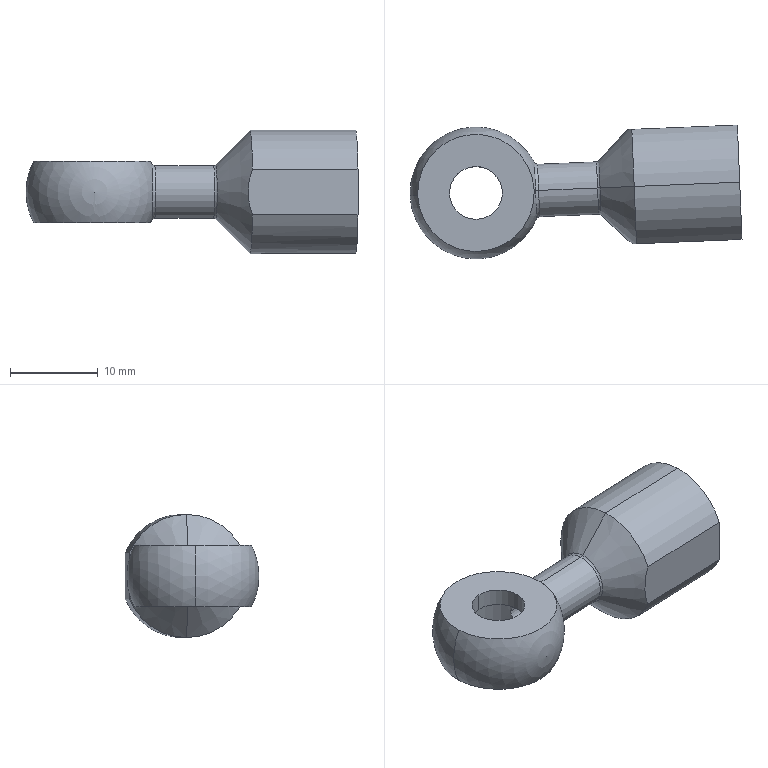Component | SolidWorks | 6.11-1937032106-0-2 | 1 solid | 33 faces | box 37.74 x 15.21 x 14 mm | volume 2451 mm3 | cylinder 16 | plane 7 | torus 4 | cone 4 | sphere 2 | commonest cylinder face diameters 6 x6 8 x3 14 x3 8.8 x2 3 x2 | material 40Cr
STEP:
#1=COLOUR_RGB('',0.7922,0.8196,0.9333);
#2=FILL_AREA_STYLE_COLOUR('',#1);
#3=FILL_AREA_STYLE('',(#2));
#4=SURFACE_STYLE_FILL_AREA(#3);
#5=SURFACE_SIDE_STYLE('',(#4));
#6=SURFACE_STYLE_USAGE(.BOTH.,#5);
#7=PRESENTATION_STYLE_ASSIGNMENT((#6));
#8=CARTESIAN_POINT('',(0.2663,-1.761,-2.076));
#9=VERTEX_POINT('',#8);
#10=CARTESIAN_POINT('',(0.2663,-1.761,-1.822));
#11=VERTEX_POINT('',#10);
#12=CARTESIAN_POINT('',(0.2663,-1.761,-1.949));
#13=DIRECTION('',(-0.9992,-0.0406,0.));
#14=DIRECTION('',(0.,0.,1.));
#15=AXIS2_PLACEMENT_3D('',#12,#13,#14);
#16=CIRCLE('',#15,0.1271);
#17=EDGE_CURVE('',#9,#11,#16,.T.);
#18=ORIENTED_EDGE('',*,*,#17,.F.);
#19=CARTESIAN_POINT('',(0.2805,-1.76,-2.067));
#20=VERTEX_POINT('',#19);
#21=CARTESIAN_POINT('',(0.2805,-1.76,-2.083));
#22=DIRECTION('',(-0.0406,0.9992,0.));
#23=DIRECTION('',(-0.9992,-0.0406,0.));
#24=AXIS2_PLACEMENT_3D('',#21,#22,#23);
#25=CIRCLE('',#24,0.01575);
#26=EDGE_CURVE('',#9,#20,#25,.T.);
#27=ORIENTED_EDGE('',*,*,#26,.T.);
#28=CARTESIAN_POINT('',(0.2805,-1.76,-1.831));
#29=VERTEX_POINT('',#28);
#30=CARTESIAN_POINT('',(0.2805,-1.76,-1.949));
#31=DIRECTION('',(0.9992,0.0406,-0.));
#32=DIRECTION('',(0.,0.,1.));
#33=AXIS2_PLACEMENT_3D('',#30,#31,#32);
#34=CIRCLE('',#33,0.1181);
#35=EDGE_CURVE('',#29,#20,#34,.T.);
#36=ORIENTED_EDGE('',*,*,#35,.F.);
#37=CARTESIAN_POINT('',(0.2805,-1.76,-1.815));
#38=DIRECTION('',(0.0406,-0.9992,0.));
#39=DIRECTION('',(0.9992,0.0406,0.));
#40=AXIS2_PLACEMENT_3D('',#37,#38,#39);
#41=CIRCLE('',#40,0.01575);
#42=EDGE_CURVE('',#11,#29,#41,.T.);
#43=ORIENTED_EDGE('',*,*,#42,.F.);
#44=EDGE_LOOP('',(#18,#27,#36,#43));
#45=FACE_OUTER_BOUND('',#44,.T.);
#46=CARTESIAN_POINT('',(0.2805,-1.76,-1.949));
#47=DIRECTION('',(-0.9992,-0.0406,0.));
#48=DIRECTION('',(0.,-0.,1.));
#49=AXIS2_PLACEMENT_3D('',#46,#47,#48);
#50=TOROIDAL_SURFACE('',#49,0.1339,0.01575);
#51=ADVANCED_FACE('',(#45),#50,.F.);
#52=CARTESIAN_POINT('',(0.5442,-1.75,-2.067));
#53=VERTEX_POINT('',#52);
#54=CARTESIAN_POINT('',(0.5442,-1.75,-1.831));
#55=VERTEX_POINT('',#54);
#56=CARTESIAN_POINT('',(0.5442,-1.75,-1.949));
#57=DIRECTION('',(-0.9992,-0.0406,0.));
#58=DIRECTION('',(0.,0.,1.));
#59=AXIS2_PLACEMENT_3D('',#56,#57,#58);
#60=CIRCLE('',#59,0.1181);
#61=EDGE_CURVE('',#53,#55,#60,.T.);
#62=ORIENTED_EDGE('',*,*,#61,.F.);
#63=CARTESIAN_POINT('',(0.5553,-1.749,-2.072));
#64=VERTEX_POINT('',#63);
#65=CARTESIAN_POINT('',(0.5442,-1.75,-2.083));
#66=DIRECTION('',(-0.0406,0.9992,0.));
#67=DIRECTION('',(-0.9992,-0.0406,0.));
#68=AXIS2_PLACEMENT_3D('',#65,#66,#67);
#69=CIRCLE('',#68,0.01575);
#70=EDGE_CURVE('',#53,#64,#69,.T.);
#71=ORIENTED_EDGE('',*,*,#70,.T.);
#72=CARTESIAN_POINT('',(0.5553,-1.749,-1.826));
#73=VERTEX_POINT('',#72);
#74=CARTESIAN_POINT('',(0.5553,-1.749,-1.949));
#75=DIRECTION('',(0.9992,0.0406,-0.));
#76=DIRECTION('',(0.,0.,-1.));
#77=AXIS2_PLACEMENT_3D('',#74,#75,#76);
#78=CIRCLE('',#77,0.1227);
#79=EDGE_CURVE('',#73,#64,#78,.T.);
#80=ORIENTED_EDGE('',*,*,#79,.F.);
#81=CARTESIAN_POINT('',(0.5442,-1.75,-1.815));
#82=DIRECTION('',(0.0406,-0.9992,0.));
#83=DIRECTION('',(0.9992,0.0406,0.));
#84=AXIS2_PLACEMENT_3D('',#81,#82,#83);
#85=CIRCLE('',#84,0.01575);
#86=EDGE_CURVE('',#55,#73,#85,.T.);
#87=ORIENTED_EDGE('',*,*,#86,.F.);
#88=EDGE_LOOP('',(#62,#71,#80,#87));
#89=FACE_OUTER_BOUND('',#88,.T.);
#90=CARTESIAN_POINT('',(0.5442,-1.75,-1.949));
#91=DIRECTION('',(-0.9992,-0.0406,0.));
#92=DIRECTION('',(0.,0.,1.));
#93=AXIS2_PLACEMENT_3D('',#90,#91,#92);
#94=TOROIDAL_SURFACE('',#93,0.1339,0.01575);
#95=ADVANCED_FACE('',(#89),#94,.F.);
#96=CARTESIAN_POINT('',(0.006394,-1.929,-1.89));
#97=VERTEX_POINT('',#96);
#98=CARTESIAN_POINT('',(-0.006394,-1.614,-1.89));
#99=VERTEX_POINT('',#98);
#100=CARTESIAN_POINT('',(0.,-1.772,-1.89));
#101=DIRECTION('',(0.,0.,-1.));
#102=DIRECTION('',(-0.0406,0.9992,0.));
#103=AXIS2_PLACEMENT_3D('',#100,#101,#102);
#104=CIRCLE('',#103,0.1575);
#105=EDGE_CURVE('',#97,#99,#104,.T.);
#106=ORIENTED_EDGE('',*,*,#105,.F.);
#107=CARTESIAN_POINT('',(0.006394,-1.929,-2.008));
#108=VERTEX_POINT('',#107);
#109=CARTESIAN_POINT('',(0.006394,-1.929,-1.89));
#110=DIRECTION('',(0.,0.,-1.));
#111=VECTOR('',#110,39.37);
#112=LINE('',#109,#111);
#113=EDGE_CURVE('',#97,#108,#112,.T.);
#114=ORIENTED_EDGE('',*,*,#113,.T.);
#115=CARTESIAN_POINT('',(-0.006394,-1.614,-2.008));
#116=VERTEX_POINT('',#115);
#117=CARTESIAN_POINT('',(0.,-1.772,-2.008));
#118=DIRECTION('',(0.,0.,-1.));
#119=DIRECTION('',(-0.0406,0.9992,0.));
#120=AXIS2_PLACEMENT_3D('',#117,#118,#119);
#121=CIRCLE('',#120,0.1575);
#122=EDGE_CURVE('',#108,#116,#121,.T.);
#123=ORIENTED_EDGE('',*,*,#122,.T.);
#124=CARTESIAN_POINT('',(-0.006394,-1.614,-1.89));
#125=DIRECTION('',(0.,0.,-1.));
#126=VECTOR('',#125,39.37);
#127=LINE('',#124,#126);
#128=EDGE_CURVE('',#99,#116,#127,.T.);
#129=ORIENTED_EDGE('',*,*,#128,.F.);
#130=EDGE_LOOP('',(#106,#114,#123,#129));
#131=FACE_OUTER_BOUND('',#130,.T.);
#132=CARTESIAN_POINT('',(0.,-1.772,-1.89));
#133=DIRECTION('',(0.,0.,-1.));
#134=DIRECTION('',(-0.0406,0.9992,0.));
#135=AXIS2_PLACEMENT_3D('',#132,#133,#134);
#136=CYLINDRICAL_SURFACE('',#135,0.1575);
#137=ADVANCED_FACE('',(#131),#136,.F.);
#138=CARTESIAN_POINT('',(0.1574,-1.765,-1.89));
#139=VERTEX_POINT('',#138);
#140=CARTESIAN_POINT('',(0.,-1.772,-1.89));
#141=DIRECTION('',(0.,0.,-1.));
#142=DIRECTION('',(-0.0406,0.9992,0.));
#143=AXIS2_PLACEMENT_3D('',#140,#141,#142);
#144=CIRCLE('',#143,0.1575);
#145=EDGE_CURVE('',#99,#139,#144,.T.);
#146=ORIENTED_EDGE('',*,*,#145,.F.);
#147=ORIENTED_EDGE('',*,*,#128,.T.);
#148=CARTESIAN_POINT('',(0.1574,-1.765,-2.008));
#149=VERTEX_POINT('',#148);
#150=CARTESIAN_POINT('',(0.,-1.772,-2.008));
#151=DIRECTION('',(0.,0.,-1.));
#152=DIRECTION('',(-0.0406,0.9992,0.));
#153=AXIS2_PLACEMENT_3D('',#150,#151,#152);
#154=CIRCLE('',#153,0.1575);
#155=EDGE_CURVE('',#116,#149,#154,.T.);
#156=ORIENTED_EDGE('',*,*,#155,.T.);
#157=CARTESIAN_POINT('',(0.1435,-1.707,-1.949));
#158=VERTEX_POINT('',#157);
#159=CARTESIAN_POINT('',(0.1435,-1.707,-1.949));
#160=CARTESIAN_POINT('',(0.1435,-1.707,-1.957));
#161=CARTESIAN_POINT('',(0.1442,-1.708,-1.964));
#162=CARTESIAN_POINT('',(0.146,-1.713,-1.975));
#163=CARTESIAN_POINT('',(0.1467,-1.714,-1.979));
#164=CARTESIAN_POINT('',(0.1483,-1.719,-1.985));
#165=CARTESIAN_POINT('',(0.1492,-1.721,-1.988));
#166=CARTESIAN_POINT('',(0.1517,-1.729,-1.996));
#167=CARTESIAN_POINT('',(0.1535,-1.736,-2.));
#168=CARTESIAN_POINT('',(0.1554,-1.746,-2.005));
#169=CARTESIAN_POINT('',(0.156,-1.75,-2.006));
#170=CARTESIAN_POINT('',(0.1569,-1.757,-2.007));
#171=CARTESIAN_POINT('',(0.1572,-1.761,-2.008));
#172=CARTESIAN_POINT('',(0.1574,-1.765,-2.008));
#173=B_SPLINE_CURVE_WITH_KNOTS('',3,(#159,#160,#161,#162,#163,#164,#165,#166,#167,#168,#169,#170,#171,#172),.UNSPECIFIED.,.F.,.F.,(4,2,2,2,2,2,4),(0.004733,0.005325,0.00562,0.005916,0.006507,0.006803,0.007099),.UNSPECIFIED.);
#174=EDGE_CURVE('',#158,#149,#173,.T.);
#175=ORIENTED_EDGE('',*,*,#174,.F.);
#176=CARTESIAN_POINT('',(0.1574,-1.765,-1.89));
#177=CARTESIAN_POINT('',(0.1572,-1.761,-1.89));
#178=CARTESIAN_POINT('',(0.1569,-1.757,-1.89));
#179=CARTESIAN_POINT('',(0.156,-1.75,-1.892));
#180=CARTESIAN_POINT('',(0.1554,-1.746,-1.893));
#181=CARTESIAN_POINT('',(0.1541,-1.739,-1.896));
#182=CARTESIAN_POINT('',(0.1533,-1.736,-1.898));
#183=CARTESIAN_POINT('',(0.1517,-1.729,-1.902));
#184=CARTESIAN_POINT('',(0.1509,-1.726,-1.904));
#185=CARTESIAN_POINT('',(0.1492,-1.721,-1.91));
#186=CARTESIAN_POINT('',(0.1483,-1.719,-1.913));
#187=CARTESIAN_POINT('',(0.1467,-1.714,-1.919));
#188=CARTESIAN_POINT('',(0.146,-1.713,-1.923));
#189=CARTESIAN_POINT('',(0.1442,-1.708,-1.933));
#190=CARTESIAN_POINT('',(0.1435,-1.707,-1.941));
#191=CARTESIAN_POINT('',(0.1435,-1.707,-1.949));
#192=B_SPLINE_CURVE_WITH_KNOTS('',3,(#176,#177,#178,#179,#180,#181,#182,#183,#184,#185,#186,#187,#188,#189,#190,#191),.UNSPECIFIED.,.F.,.F.,(4,2,2,2,2,2,2,4),(0.002367,0.002663,0.002959,0.003255,0.00355,0.003846,0.004142,0.004733),.UNSPECIFIED.);
#193=EDGE_CURVE('',#139,#158,#192,.T.);
#194=ORIENTED_EDGE('',*,*,#193,.F.);
#195=EDGE_LOOP('',(#146,#147,#156,#175,#194));
#196=FACE_OUTER_BOUND('',#195,.T.);
#197=CARTESIAN_POINT('',(0.,-1.772,-1.89));
#198=DIRECTION('',(0.,0.,-1.));
#199=DIRECTION('',(-0.0406,0.9992,0.));
#200=AXIS2_PLACEMENT_3D('',#197,#198,#199);
#201=CYLINDRICAL_SURFACE('',#200,0.1575);
#202=ADVANCED_FACE('',(#196),#201,.F.);
#203=CARTESIAN_POINT('',(0.7797,-1.567,-1.949));
#204=VERTEX_POINT('',#203);
#205=CARTESIAN_POINT('',(0.7938,-1.913,-1.949));
#206=VERTEX_POINT('',#205);
#207=CARTESIAN_POINT('',(0.7868,-1.74,-1.949));
#208=DIRECTION('',(0.9992,0.0406,0.));
#209=DIRECTION('',(0.0406,-0.9992,0.));
#210=AXIS2_PLACEMENT_3D('',#207,#208,#209);
#211=CIRCLE('',#210,0.1732);
#212=EDGE_CURVE('',#204,#206,#211,.T.);
#213=ORIENTED_EDGE('',*,*,#212,.F.);
#214=CARTESIAN_POINT('',(1.173,-1.551,-1.949));
#215=VERTEX_POINT('',#214);
#216=CARTESIAN_POINT('',(1.173,-1.551,-1.949));
#217=DIRECTION('',(0.9992,0.0406,0.));
#218=VECTOR('',#217,39.37);
#219=LINE('',#216,#218);
#220=EDGE_CURVE('',#204,#215,#219,.T.);
#221=ORIENTED_EDGE('',*,*,#220,.T.);
#222=CARTESIAN_POINT('',(1.187,-1.897,-1.949));
#223=VERTEX_POINT('',#222);
#224=CARTESIAN_POINT('',(1.18,-1.724,-1.949));
#225=DIRECTION('',(0.9992,0.0406,0.));
#226=DIRECTION('',(0.0406,-0.9992,0.));
#227=AXIS2_PLACEMENT_3D('',#224,#225,#226);
#228=CIRCLE('',#227,0.1732);
#229=EDGE_CURVE('',#215,#223,#228,.T.);
#230=ORIENTED_EDGE('',*,*,#229,.T.);
#231=CARTESIAN_POINT('',(1.187,-1.897,-1.949));
#232=DIRECTION('',(0.9992,0.0406,0.));
#233=VECTOR('',#232,39.37);
#234=LINE('',#231,#233);
#235=EDGE_CURVE('',#206,#223,#234,.T.);
#236=ORIENTED_EDGE('',*,*,#235,.F.);
#237=EDGE_LOOP('',(#213,#221,#230,#236));
#238=FACE_OUTER_BOUND('',#237,.T.);
#239=CARTESIAN_POINT('',(1.18,-1.724,-1.949));
#240=DIRECTION('',(0.9992,0.0406,0.));
#241=DIRECTION('',(0.0406,-0.9992,0.));
#242=AXIS2_PLACEMENT_3D('',#239,#240,#241);
#243=CYLINDRICAL_SURFACE('',#242,0.1732);
#244=ADVANCED_FACE('',(#238),#243,.F.);
#245=CARTESIAN_POINT('',(0.7158,-1.683,-1.949));
#246=VERTEX_POINT('',#245);
#247=CARTESIAN_POINT('',(0.7206,-1.801,-1.949));
#248=VERTEX_POINT('',#247);
#249=CARTESIAN_POINT('',(0.7182,-1.742,-1.949));
#250=DIRECTION('',(0.9992,0.0406,0.));
#251=DIRECTION('',(0.0406,-0.9992,0.));
#252=AXIS2_PLACEMENT_3D('',#249,#250,#251);
#253=CIRCLE('',#252,0.05906);
#254=EDGE_CURVE('',#246,#248,#253,.T.);
#255=ORIENTED_EDGE('',*,*,#254,.F.);
#256=CARTESIAN_POINT('',(0.7797,-1.567,-1.949));
#257=DIRECTION('',(0.4798,0.8774,-0.));
#258=VECTOR('',#257,39.37);
#259=LINE('',#256,#258);
#260=EDGE_CURVE('',#246,#204,#259,.T.);
#261=ORIENTED_EDGE('',*,*,#260,.T.);
#262=ORIENTED_EDGE('',*,*,#212,.T.);
#263=CARTESIAN_POINT('',(0.7938,-1.913,-1.949));
#264=DIRECTION('',(0.5494,-0.8355,0.));
#265=VECTOR('',#264,39.37);
#266=LINE('',#263,#265);
#267=EDGE_CURVE('',#248,#206,#266,.T.);
#268=ORIENTED_EDGE('',*,*,#267,.F.);
#269=EDGE_LOOP('',(#255,#261,#262,#268));
#270=FACE_OUTER_BOUND('',#269,.T.);
#271=CARTESIAN_POINT('',(0.7868,-1.74,-1.949));
#272=DIRECTION('',(0.9992,0.0406,0.));
#273=DIRECTION('',(0.0406,-0.9992,0.));
#274=AXIS2_PLACEMENT_3D('',#271,#272,#273);
#275=CONICAL_SURFACE('',#274,0.1732,1.03);
#276=ADVANCED_FACE('',(#270),#275,.F.);
#277=ORIENTED_EDGE('',*,*,#193,.T.);
#278=CARTESIAN_POINT('',(1.178,-1.665,-1.949));
#279=DIRECTION('',(0.9992,0.0406,0.));
#280=VECTOR('',#279,39.37);
#281=LINE('',#278,#280);
#282=EDGE_CURVE('',#158,#246,#281,.T.);
#283=ORIENTED_EDGE('',*,*,#282,.T.);
#284=ORIENTED_EDGE('',*,*,#254,.T.);
#285=CARTESIAN_POINT('',(0.1483,-1.825,-1.949));
#286=VERTEX_POINT('',#285);
#287=CARTESIAN_POINT('',(1.183,-1.783,-1.949));
#288=DIRECTION('',(0.9992,0.0406,0.));
#289=VECTOR('',#288,39.37);
#290=LINE('',#287,#289);
#291=EDGE_CURVE('',#286,#248,#290,.T.);
#292=ORIENTED_EDGE('',*,*,#291,.F.);
#293=CARTESIAN_POINT('',(0.1483,-1.825,-1.949));
#294=CARTESIAN_POINT('',(0.1483,-1.825,-1.945));
#295=CARTESIAN_POINT('',(0.1484,-1.824,-1.941));
#296=CARTESIAN_POINT('',(0.1489,-1.823,-1.933));
#297=CARTESIAN_POINT('',(0.1494,-1.822,-1.93));
#298=CARTESIAN_POINT('',(0.1508,-1.817,-1.919));
#299=CARTESIAN_POINT('',(0.1522,-1.813,-1.912));
#300=CARTESIAN_POINT('',(0.1547,-1.802,-1.902));
#301=CARTESIAN_POINT('',(0.1559,-1.795,-1.897));
#302=CARTESIAN_POINT('',(0.157,-1.784,-1.893));
#303=CARTESIAN_POINT('',(0.1573,-1.781,-1.892));
#304=CARTESIAN_POINT('',(0.1575,-1.773,-1.89));
#305=CARTESIAN_POINT('',(0.1575,-1.769,-1.89));
#306=CARTESIAN_POINT('',(0.1574,-1.765,-1.89));
#307=B_SPLINE_CURVE_WITH_KNOTS('',3,(#293,#294,#295,#296,#297,#298,#299,#300,#301,#302,#303,#304,#305,#306),.UNSPECIFIED.,.F.,.F.,(4,2,2,2,2,2,4),(0.,0.0002959,0.0005918,0.001184,0.001775,0.002071,0.002367),.UNSPECIFIED.);
#308=EDGE_CURVE('',#286,#139,#307,.T.);
#309=ORIENTED_EDGE('',*,*,#308,.T.);
#310=EDGE_LOOP('',(#277,#283,#284,#292,#309));
#311=FACE_OUTER_BOUND('',#310,.T.);
#312=CARTESIAN_POINT('',(1.18,-1.724,-1.949));
#313=DIRECTION('',(0.9992,0.0406,0.));
#314=DIRECTION('',(0.0406,-0.9992,0.));
#315=AXIS2_PLACEMENT_3D('',#312,#313,#314);
#316=CYLINDRICAL_SURFACE('',#315,0.05906);
#317=ADVANCED_FACE('',(#311),#316,.F.);
#318=CARTESIAN_POINT('',(-0.004795,-1.654,-2.008));
#319=VERTEX_POINT('',#318);
#320=CARTESIAN_POINT('',(0.004795,-1.89,-2.008));
#321=VERTEX_POINT('',#320);
#322=CARTESIAN_POINT('',(0.,-1.772,-2.008));
#323=DIRECTION('',(0.,0.,1.));
#324=DIRECTION('',(-0.0406,0.9992,0.));
#325=AXIS2_PLACEMENT_3D('',#322,#323,#324);
#326=CIRCLE('',#325,0.1181);
#327=EDGE_CURVE('',#319,#321,#326,.T.);
#328=ORIENTED_EDGE('',*,*,#327,.T.);
#329=CARTESIAN_POINT('',(0.004795,-1.89,-2.087));
#330=VERTEX_POINT('',#329);
#331=CARTESIAN_POINT('',(0.004795,-1.89,-2.087));
#332=DIRECTION('',(0.,0.,-1.));
#333=VECTOR('',#332,39.37);
#334=LINE('',#331,#333);
#335=EDGE_CURVE('',#321,#330,#334,.T.);
#336=ORIENTED_EDGE('',*,*,#335,.T.);
#337=CARTESIAN_POINT('',(-0.004795,-1.654,-2.087));
#338=VERTEX_POINT('',#337);
#339=CARTESIAN_POINT('',(0.,-1.772,-2.087));
#340=DIRECTION('',(0.,0.,-1.));
#341=DIRECTION('',(-0.0406,0.9992,0.));
#342=AXIS2_PLACEMENT_3D('',#339,#340,#341);
#343=CIRCLE('',#342,0.1181);
#344=EDGE_CURVE('',#330,#338,#343,.T.);
#345=ORIENTED_EDGE('',*,*,#344,.T.);
#346=CARTESIAN_POINT('',(-0.004795,-1.654,-2.087));
#347=DIRECTION('',(0.,0.,-1.));
#348=VECTOR('',#347,39.37);
#349=LINE('',#346,#348);
#350=EDGE_CURVE('',#319,#338,#349,.T.);
#351=ORIENTED_EDGE('',*,*,#350,.F.);
#352=EDGE_LOOP('',(#328,#336,#345,#351));
#353=FACE_OUTER_BOUND('',#352,.T.);
#354=CARTESIAN_POINT('',(0.,-1.772,-2.087));
#355=DIRECTION('',(0.,0.,-1.));
#356=DIRECTION('',(-0.0406,0.9992,0.));
#357=AXIS2_PLACEMENT_3D('',#354,#355,#356);
#358=CYLINDRICAL_SURFACE('',#357,0.1181);
#359=ADVANCED_FACE('',(#353),#358,.F.);
#360=CARTESIAN_POINT('',(0.5442,-1.75,-1.949));
#361=DIRECTION('',(-0.9992,-0.0406,0.));
#362=DIRECTION('',(0.,0.,1.));
#363=AXIS2_PLACEMENT_3D('',#360,#361,#362);
#364=CIRCLE('',#363,0.1181);
#365=EDGE_CURVE('',#55,#53,#364,.T.);
#366=ORIENTED_EDGE('',*,*,#365,.T.);
#367=CARTESIAN_POINT('',(-0.295,-1.784,-2.067));
#368=DIRECTION('',(-0.9992,-0.0406,0.));
#369=VECTOR('',#368,39.37);
#370=LINE('',#367,#369);
#371=EDGE_CURVE('',#53,#20,#370,.T.);
#372=ORIENTED_EDGE('',*,*,#371,.T.);
#373=CARTESIAN_POINT('',(0.2805,-1.76,-1.949));
#374=DIRECTION('',(0.9992,0.0406,-0.));
#375=DIRECTION('',(0.,0.,1.));
#376=AXIS2_PLACEMENT_3D('',#373,#374,#375);
#377=CIRCLE('',#376,0.1181);
#378=EDGE_CURVE('',#20,#29,#377,.T.);
#379=ORIENTED_EDGE('',*,*,#378,.T.);
#380=CARTESIAN_POINT('',(-0.295,-1.784,-1.831));
#381=DIRECTION('',(-0.9992,-0.0406,0.));
#382=VECTOR('',#381,39.37);
#383=LINE('',#380,#382);
#384=EDGE_CURVE('',#55,#29,#383,.T.);
#385=ORIENTED_EDGE('',*,*,#384,.F.);
#386=EDGE_LOOP('',(#366,#372,#379,#385));
#387=FACE_OUTER_BOUND('',#386,.T.);
#388=CARTESIAN_POINT('',(-0.295,-1.784,-1.949));
#389=DIRECTION('',(-0.9992,-0.0406,0.));
#390=DIRECTION('',(0.,0.,1.));
#391=AXIS2_PLACEMENT_3D('',#388,#389,#390);
#392=CYLINDRICAL_SURFACE('',#391,0.1181);
#393=ADVANCED_FACE('',(#387),#392,.T.);
#394=ORIENTED_EDGE('',*,*,#17,.T.);
#395=CARTESIAN_POINT('',(0.2609,-1.761,-1.811));
#396=VERTEX_POINT('',#395);
#397=CARTESIAN_POINT('',(0.,-1.772,-1.949));
#398=DIRECTION('',(0.0406,-0.9992,-0.));
#399=DIRECTION('',(0.9992,0.0406,0.));
#400=AXIS2_PLACEMENT_3D('',#397,#398,#399);
#401=CIRCLE('',#400,0.2953);
#402=EDGE_CURVE('',#11,#396,#401,.T.);
#403=ORIENTED_EDGE('',*,*,#402,.T.);
#404=CARTESIAN_POINT('',(-0.2609,-1.782,-1.811));
#405=VERTEX_POINT('',#404);
#406=CARTESIAN_POINT('',(0.,-1.772,-1.811));
#407=DIRECTION('',(0.,0.,-1.));
#408=DIRECTION('',(-0.0406,0.9992,0.));
#409=AXIS2_PLACEMENT_3D('',#406,#407,#408);
#410=CIRCLE('',#409,0.2612);
#411=EDGE_CURVE('',#396,#405,#410,.T.);
#412=ORIENTED_EDGE('',*,*,#411,.T.);
#413=CARTESIAN_POINT('',(-0.295,-1.784,-1.949));
#414=VERTEX_POINT('',#413);
#415=CARTESIAN_POINT('',(0.,-1.772,-1.949));
#416=DIRECTION('',(0.0406,-0.9992,-0.));
#417=DIRECTION('',(0.9992,0.0406,0.));
#418=AXIS2_PLACEMENT_3D('',#415,#416,#417);
#419=CIRCLE('',#418,0.2953);
#420=EDGE_CURVE('',#405,#414,#419,.T.);
#421=ORIENTED_EDGE('',*,*,#420,.T.);
#422=CARTESIAN_POINT('',(-0.2609,-1.782,-2.087));
#423=VERTEX_POINT('',#422);
#424=CARTESIAN_POINT('',(0.,-1.772,-1.949));
#425=DIRECTION('',(-0.0406,0.9992,0.));
#426=DIRECTION('',(-0.9992,-0.0406,0.));
#427=AXIS2_PLACEMENT_3D('',#424,#425,#426);
#428=CIRCLE('',#427,0.2953);
#429=EDGE_CURVE('',#423,#414,#428,.T.);
#430=ORIENTED_EDGE('',*,*,#429,.F.);
#431=CARTESIAN_POINT('',(0.2609,-1.761,-2.087));
#432=VERTEX_POINT('',#431);
#433=CARTESIAN_POINT('',(0.,-1.772,-2.087));
#434=DIRECTION('',(0.,0.,1.));
#435=DIRECTION('',(0.0406,-0.9992,0.));
#436=AXIS2_PLACEMENT_3D('',#433,#434,#435);
#437=CIRCLE('',#436,0.2612);
#438=EDGE_CURVE('',#423,#432,#437,.T.);
#439=ORIENTED_EDGE('',*,*,#438,.T.);
#440=CARTESIAN_POINT('',(0.,-1.772,-1.949));
#441=DIRECTION('',(-0.0406,0.9992,0.));
#442=DIRECTION('',(-0.9992,-0.0406,0.));
#443=AXIS2_PLACEMENT_3D('',#440,#441,#442);
#444=CIRCLE('',#443,0.2953);
#445=EDGE_CURVE('',#9,#432,#444,.T.);
#446=ORIENTED_EDGE('',*,*,#445,.F.);
#447=EDGE_LOOP('',(#394,#403,#412,#421,#430,#439,#446));
#448=FACE_OUTER_BOUND('',#447,.T.);
#449=CARTESIAN_POINT('',(0.,-1.772,-1.949));
#450=DIRECTION('',(0.0406,-0.9992,-0.));
#451=DIRECTION('',(-0.,0.,-1.));
#452=AXIS2_PLACEMENT_3D('',#449,#450,#451);
#453=SPHERICAL_SURFACE('',#452,0.2953);
#454=ADVANCED_FACE('',(#448),#453,.T.);
#455=CARTESIAN_POINT('',(0.004795,-1.89,-1.811));
#456=VERTEX_POINT('',#455);
#457=CARTESIAN_POINT('',(-0.004795,-1.654,-1.811));
#458=VERTEX_POINT('',#457);
#459=CARTESIAN_POINT('',(0.,-1.772,-1.811));
#460=DIRECTION('',(0.,0.,-1.));
#461=DIRECTION('',(-0.0406,0.9992,0.));
#462=AXIS2_PLACEMENT_3D('',#459,#460,#461);
#463=CIRCLE('',#462,0.1181);
#464=EDGE_CURVE('',#456,#458,#463,.T.);
#465=ORIENTED_EDGE('',*,*,#464,.F.);
#466=CARTESIAN_POINT('',(0.004795,-1.89,-1.89));
#467=VERTEX_POINT('',#466);
#468=CARTESIAN_POINT('',(0.004795,-1.89,-2.087));
#469=DIRECTION('',(0.,0.,-1.));
#470=VECTOR('',#469,39.37);
#471=LINE('',#468,#470);
#472=EDGE_CURVE('',#456,#467,#471,.T.);
#473=ORIENTED_EDGE('',*,*,#472,.T.);
#474=CARTESIAN_POINT('',(-0.004795,-1.654,-1.89));
#475=VERTEX_POINT('',#474);
#476=CARTESIAN_POINT('',(0.,-1.772,-1.89));
#477=DIRECTION('',(0.,0.,1.));
#478=DIRECTION('',(-0.0406,0.9992,0.));
#479=AXIS2_PLACEMENT_3D('',#476,#477,#478);
#480=CIRCLE('',#479,0.1181);
#481=EDGE_CURVE('',#475,#467,#480,.T.);
#482=ORIENTED_EDGE('',*,*,#481,.F.);
#483=CARTESIAN_POINT('',(-0.004795,-1.654,-2.087));
#484=DIRECTION('',(0.,0.,-1.));
#485=VECTOR('',#484,39.37);
#486=LINE('',#483,#485);
#487=EDGE_CURVE('',#458,#475,#486,.T.);
#488=ORIENTED_EDGE('',*,*,#487,.F.);
#489=EDGE_LOOP('',(#465,#473,#482,#488));
#490=FACE_OUTER_BOUND('',#489,.T.);
#491=CARTESIAN_POINT('',(0.,-1.772,-2.087));
#492=DIRECTION('',(0.,0.,-1.));
#493=DIRECTION('',(-0.0406,0.9992,0.));
#494=AXIS2_PLACEMENT_3D('',#491,#492,#493);
#495=CYLINDRICAL_SURFACE('',#494,0.1181);
#496=ADVANCED_FACE('',(#490),#495,.F.);
#497=CARTESIAN_POINT('',(1.191,-1.979,-1.847));
#498=VERTEX_POINT('',#497);
#499=CARTESIAN_POINT('',(1.18,-1.724,-1.673));
#500=VERTEX_POINT('',#499);
#501=CARTESIAN_POINT('',(1.18,-1.724,-1.949));
#502=DIRECTION('',(-0.9992,-0.0406,0.));
#503=DIRECTION('',(0.,0.,1.));
#504=AXIS2_PLACEMENT_3D('',#501,#502,#503);
#505=CIRCLE('',#504,0.2756);
#506=EDGE_CURVE('',#498,#500,#505,.T.);
#507=ORIENTED_EDGE('',*,*,#506,.T.);
#508=CARTESIAN_POINT('',(0.7081,-1.743,-1.673));
#509=VERTEX_POINT('',#508);
#510=CARTESIAN_POINT('',(-0.295,-1.784,-1.673));
#511=DIRECTION('',(-0.9992,-0.0406,0.));
#512=VECTOR('',#511,39.37);
#513=LINE('',#510,#512);
#514=EDGE_CURVE('',#500,#509,#513,.T.);
#515=ORIENTED_EDGE('',*,*,#514,.T.);
#516=CARTESIAN_POINT('',(0.7185,-1.999,-1.847));
#517=VERTEX_POINT('',#516);
#518=CARTESIAN_POINT('',(0.7081,-1.743,-1.949));
#519=DIRECTION('',(-0.9992,-0.0406,0.));
#520=DIRECTION('',(0.,0.,1.));
#521=AXIS2_PLACEMENT_3D('',#518,#519,#520);
#522=CIRCLE('',#521,0.2756);
#523=EDGE_CURVE('',#517,#509,#522,.T.);
#524=ORIENTED_EDGE('',*,*,#523,.F.);
#525=CARTESIAN_POINT('',(-0.2846,-2.039,-1.847));
#526=DIRECTION('',(-0.9992,-0.0406,0.));
#527=VECTOR('',#526,39.37);
#528=LINE('',#525,#527);
#529=EDGE_CURVE('',#498,#517,#528,.T.);
#530=ORIENTED_EDGE('',*,*,#529,.F.);
#531=EDGE_LOOP('',(#507,#515,#524,#530));
#532=FACE_OUTER_BOUND('',#531,.T.);
#533=CARTESIAN_POINT('',(-0.295,-1.784,-1.949));
#534=DIRECTION('',(-0.9992,-0.0406,0.));
#535=DIRECTION('',(0.,0.,1.));
#536=AXIS2_PLACEMENT_3D('',#533,#534,#535);
#537=CYLINDRICAL_SURFACE('',#536,0.2756);
#538=ADVANCED_FACE('',(#532),#537,.T.);
#539=CARTESIAN_POINT('',(0.5553,-1.749,-1.949));
#540=DIRECTION('',(0.9992,0.0406,-0.));
#541=DIRECTION('',(0.,0.,-1.));
#542=AXIS2_PLACEMENT_3D('',#539,#540,#541);
#543=CIRCLE('',#542,0.1227);
#544=EDGE_CURVE('',#64,#73,#543,.T.);
#545=ORIENTED_EDGE('',*,*,#544,.T.);
#546=CARTESIAN_POINT('',(0.7081,-1.743,-1.673));
#547=DIRECTION('',(0.7065,0.02871,0.7071));
#548=VECTOR('',#547,39.37);
#549=LINE('',#546,#548);
#550=EDGE_CURVE('',#73,#509,#549,.T.);
#551=ORIENTED_EDGE('',*,*,#550,.T.);
#552=CARTESIAN_POINT('',(0.6977,-1.487,-1.847));
#553=VERTEX_POINT('',#552);
#554=CARTESIAN_POINT('',(0.7081,-1.743,-1.949));
#555=DIRECTION('',(-0.9992,-0.0406,0.));
#556=DIRECTION('',(0.,0.,1.));
#557=AXIS2_PLACEMENT_3D('',#554,#555,#556);
#558=CIRCLE('',#557,0.2756);
#559=EDGE_CURVE('',#509,#553,#558,.T.);
#560=ORIENTED_EDGE('',*,*,#559,.T.);
#561=CARTESIAN_POINT('',(0.6977,-1.487,-2.051));
#562=VERTEX_POINT('',#561);
#563=CARTESIAN_POINT('',(0.6977,-1.487,-2.051));
#564=CARTESIAN_POINT('',(0.6947,-1.487,-2.043));
#565=CARTESIAN_POINT('',(0.6919,-1.487,-2.035));
#566=CARTESIAN_POINT('',(0.687,-1.488,-2.018));
#567=CARTESIAN_POINT('',(0.6849,-1.488,-2.009));
#568=CARTESIAN_POINT('',(0.6799,-1.488,-1.984));
#569=CARTESIAN_POINT('',(0.678,-1.488,-1.967));
#570=CARTESIAN_POINT('',(0.678,-1.488,-1.94));
#571=CARTESIAN_POINT('',(0.6785,-1.488,-1.931));
#572=CARTESIAN_POINT('',(0.6802,-1.488,-1.914));
#573=CARTESIAN_POINT('',(0.6815,-1.488,-1.905));
#574=CARTESIAN_POINT('',(0.6866,-1.488,-1.88));
#575=CARTESIAN_POINT('',(0.6916,-1.487,-1.863));
#576=CARTESIAN_POINT('',(0.6977,-1.487,-1.847));
#577=B_SPLINE_CURVE_WITH_KNOTS('',3,(#563,#564,#565,#566,#567,#568,#569,#570,#571,#572,#573,#574,#575,#576),.UNSPECIFIED.,.F.,.F.,(4,2,2,2,2,2,4),(0.02679,0.02744,0.0281,0.02942,0.03008,0.03073,0.03205),.UNSPECIFIED.);
#578=EDGE_CURVE('',#562,#553,#577,.T.);
#579=ORIENTED_EDGE('',*,*,#578,.F.);
#580=CARTESIAN_POINT('',(0.7081,-1.743,-2.224));
#581=VERTEX_POINT('',#580);
#582=CARTESIAN_POINT('',(0.7081,-1.743,-1.949));
#583=DIRECTION('',(-0.9992,-0.0406,0.));
#584=DIRECTION('',(0.,0.,1.));
#585=AXIS2_PLACEMENT_3D('',#582,#583,#584);
#586=CIRCLE('',#585,0.2756);
#587=EDGE_CURVE('',#562,#581,#586,.T.);
#588=ORIENTED_EDGE('',*,*,#587,.T.);
#589=CARTESIAN_POINT('',(0.7081,-1.743,-2.224));
#590=DIRECTION('',(0.7065,0.02871,-0.7071));
#591=VECTOR('',#590,39.37);
#592=LINE('',#589,#591);
#593=EDGE_CURVE('',#64,#581,#592,.T.);
#594=ORIENTED_EDGE('',*,*,#593,.F.);
#595=EDGE_LOOP('',(#545,#551,#560,#579,#588,#594));
#596=FACE_OUTER_BOUND('',#595,.T.);
#597=CARTESIAN_POINT('',(0.7081,-1.743,-1.949));
#598=DIRECTION('',(0.9992,0.0406,-0.));
#599=DIRECTION('',(0.,0.,-1.));
#600=AXIS2_PLACEMENT_3D('',#597,#598,#599);
#601=CONICAL_SURFACE('',#600,0.2756,0.7854);
#602=ADVANCED_FACE('',(#596),#601,.T.);
#603=ORIENTED_EDGE('',*,*,#550,.F.);
#604=ORIENTED_EDGE('',*,*,#79,.T.);
#605=ORIENTED_EDGE('',*,*,#593,.T.);
#606=CARTESIAN_POINT('',(0.7185,-1.999,-2.051));
#607=VERTEX_POINT('',#606);
#608=CARTESIAN_POINT('',(0.7081,-1.743,-1.949));
#609=DIRECTION('',(-0.9992,-0.0406,0.));
#610=DIRECTION('',(0.,0.,1.));
#611=AXIS2_PLACEMENT_3D('',#608,#609,#610);
#612=CIRCLE('',#611,0.2756);
#613=EDGE_CURVE('',#581,#607,#612,.T.);
#614=ORIENTED_EDGE('',*,*,#613,.T.);
#615=CARTESIAN_POINT('',(0.7185,-1.999,-1.847));
#616=CARTESIAN_POINT('',(0.7124,-1.999,-1.863));
#617=CARTESIAN_POINT('',(0.7074,-1.999,-1.88));
#618=CARTESIAN_POINT('',(0.7023,-1.999,-1.905));
#619=CARTESIAN_POINT('',(0.701,-1.999,-1.914));
#620=CARTESIAN_POINT('',(0.6992,-1.999,-1.931));
#621=CARTESIAN_POINT('',(0.6988,-1.999,-1.94));
#622=CARTESIAN_POINT('',(0.6988,-1.999,-1.967));
#623=CARTESIAN_POINT('',(0.7006,-1.999,-1.984));
#624=CARTESIAN_POINT('',(0.7057,-1.999,-2.009));
#625=CARTESIAN_POINT('',(0.7078,-1.999,-2.018));
#626=CARTESIAN_POINT('',(0.7127,-1.999,-2.035));
#627=CARTESIAN_POINT('',(0.7154,-1.999,-2.043));
#628=CARTESIAN_POINT('',(0.7185,-1.999,-2.051));
#629=B_SPLINE_CURVE_WITH_KNOTS('',3,(#615,#616,#617,#618,#619,#620,#621,#622,#623,#624,#625,#626,#627,#628),.UNSPECIFIED.,.F.,.F.,(4,2,2,2,2,2,4),(0.0245,0.02582,0.02647,0.02713,0.02844,0.02909,0.02975),.UNSPECIFIED.);
#630=EDGE_CURVE('',#517,#607,#629,.T.);
#631=ORIENTED_EDGE('',*,*,#630,.F.);
#632=ORIENTED_EDGE('',*,*,#523,.T.);
#633=EDGE_LOOP('',(#603,#604,#605,#614,#631,#632));
#634=FACE_OUTER_BOUND('',#633,.T.);
#635=CARTESIAN_POINT('',(0.7081,-1.743,-1.949));
#636=DIRECTION('',(0.9992,0.0406,-0.));
#637=DIRECTION('',(0.,0.,-1.));
#638=AXIS2_PLACEMENT_3D('',#635,#636,#637);
#639=CONICAL_SURFACE('',#638,0.2756,0.7854);
#640=ADVANCED_FACE('',(#634),#639,.T.);
#641=ORIENTED_EDGE('',*,*,#514,.F.);
#642=CARTESIAN_POINT('',(1.17,-1.468,-1.847));
#643=VERTEX_POINT('',#642);
#644=CARTESIAN_POINT('',(1.18,-1.724,-1.949));
#645=DIRECTION('',(-0.9992,-0.0406,0.));
#646=DIRECTION('',(0.,0.,1.));
#647=AXIS2_PLACEMENT_3D('',#644,#645,#646);
#648=CIRCLE('',#647,0.2756);
#649=EDGE_CURVE('',#500,#643,#648,.T.);
#650=ORIENTED_EDGE('',*,*,#649,.T.);
#651=CARTESIAN_POINT('',(-0.3054,-1.528,-1.847));
#652=DIRECTION('',(0.9992,0.0406,-0.));
#653=VECTOR('',#652,39.37);
#654=LINE('',#651,#653);
#655=EDGE_CURVE('',#553,#643,#654,.T.);
#656=ORIENTED_EDGE('',*,*,#655,.F.);
#657=ORIENTED_EDGE('',*,*,#559,.F.);
#658=EDGE_LOOP('',(#641,#650,#656,#657));
#659=FACE_OUTER_BOUND('',#658,.T.);
#660=CARTESIAN_POINT('',(-0.295,-1.784,-1.949));
#661=DIRECTION('',(-0.9992,-0.0406,0.));
#662=DIRECTION('',(0.,0.,1.));
#663=AXIS2_PLACEMENT_3D('',#660,#661,#662);
#664=CYLINDRICAL_SURFACE('',#663,0.2756);
#665=ADVANCED_FACE('',(#659),#664,.T.);
#666=CARTESIAN_POINT('',(1.191,-1.979,-2.051));
#667=VERTEX_POINT('',#666);
#668=CARTESIAN_POINT('',(-0.2846,-2.039,-2.051));
#669=DIRECTION('',(0.9992,0.0406,-0.));
#670=VECTOR('',#669,39.37);
#671=LINE('',#668,#670);
#672=EDGE_CURVE('',#607,#667,#671,.T.);
#673=ORIENTED_EDGE('',*,*,#672,.F.);
#674=ORIENTED_EDGE('',*,*,#613,.F.);
#675=ORIENTED_EDGE('',*,*,#587,.F.);
#676=CARTESIAN_POINT('',(1.17,-1.468,-2.051));
#677=VERTEX_POINT('',#676);
#678=CARTESIAN_POINT('',(-0.3054,-1.528,-2.051));
#679=DIRECTION('',(-0.9992,-0.0406,0.));
#680=VECTOR('',#679,39.37);
#681=LINE('',#678,#680);
#682=EDGE_CURVE('',#677,#562,#681,.T.);
#683=ORIENTED_EDGE('',*,*,#682,.F.);
#684=CARTESIAN_POINT('',(1.18,-1.724,-1.949));
#685=DIRECTION('',(-0.9992,-0.0406,0.));
#686=DIRECTION('',(0.,0.,1.));
#687=AXIS2_PLACEMENT_3D('',#684,#685,#686);
#688=CIRCLE('',#687,0.2756);
#689=EDGE_CURVE('',#677,#667,#688,.T.);
#690=ORIENTED_EDGE('',*,*,#689,.T.);
#691=EDGE_LOOP('',(#673,#674,#675,#683,#690));
#692=FACE_OUTER_BOUND('',#691,.T.);
#693=CARTESIAN_POINT('',(-0.295,-1.784,-1.949));
#694=DIRECTION('',(-0.9992,-0.0406,0.));
#695=DIRECTION('',(0.,0.,1.));
#696=AXIS2_PLACEMENT_3D('',#693,#694,#695);
#697=CYLINDRICAL_SURFACE('',#696,0.2756);
#698=ADVANCED_FACE('',(#692),#697,.T.);
#699=CARTESIAN_POINT('',(1.18,-1.724,-1.949));
#700=DIRECTION('',(0.9992,0.0406,0.));
#701=DIRECTION('',(0.0406,-0.9992,0.));
#702=AXIS2_PLACEMENT_3D('',#699,#700,#701);
#703=CIRCLE('',#702,0.1732);
#704=EDGE_CURVE('',#223,#215,#703,.T.);
#705=ORIENTED_EDGE('',*,*,#704,.F.);
#706=ORIENTED_EDGE('',*,*,#229,.F.);
#707=EDGE_LOOP('',(#705,#706));
#708=FACE_BOUND('',#707,.T.);
#709=CARTESIAN_POINT('',(1.191,-1.979,-2.224));
#710=DIRECTION('',(0.,-0.,1.));
#711=VECTOR('',#710,39.37);
#712=LINE('',#709,#711);
#713=EDGE_CURVE('',#667,#498,#712,.T.);
#714=ORIENTED_EDGE('',*,*,#713,.F.);
#715=ORIENTED_EDGE('',*,*,#689,.F.);
#716=CARTESIAN_POINT('',(1.17,-1.468,-2.224));
#717=DIRECTION('',(-0.,0.,-1.));
#718=VECTOR('',#717,39.37);
#719=LINE('',#716,#718);
#720=EDGE_CURVE('',#643,#677,#719,.T.);
#721=ORIENTED_EDGE('',*,*,#720,.F.);
#722=ORIENTED_EDGE('',*,*,#649,.F.);
#723=ORIENTED_EDGE('',*,*,#506,.F.);
#724=EDGE_LOOP('',(#714,#715,#721,#722,#723));
#725=FACE_OUTER_BOUND('',#724,.T.);
#726=CARTESIAN_POINT('',(1.18,-1.724,-2.224));
#727=DIRECTION('',(-0.9992,-0.0406,0.));
#728=DIRECTION('',(0.,0.,1.));
#729=AXIS2_PLACEMENT_3D('',#726,#727,#728);
#730=PLANE('',#729);
#731=ADVANCED_FACE('',(#708,#725),#730,.F.);
#732=ORIENTED_EDGE('',*,*,#472,.F.);
#733=CARTESIAN_POINT('',(0.,-1.772,-1.811));
#734=DIRECTION('',(0.,0.,-1.));
#735=DIRECTION('',(-0.0406,0.9992,0.));
#736=AXIS2_PLACEMENT_3D('',#733,#734,#735);
#737=CIRCLE('',#736,0.1181);
#738=EDGE_CURVE('',#458,#456,#737,.T.);
#739=ORIENTED_EDGE('',*,*,#738,.F.);
#740=ORIENTED_EDGE('',*,*,#487,.T.);
#741=CARTESIAN_POINT('',(0.,-1.772,-1.89));
#742=DIRECTION('',(0.,0.,1.));
#743=DIRECTION('',(-0.0406,0.9992,0.));
#744=AXIS2_PLACEMENT_3D('',#741,#742,#743);
#745=CIRCLE('',#744,0.1181);
#746=EDGE_CURVE('',#467,#475,#745,.T.);
#747=ORIENTED_EDGE('',*,*,#746,.F.);
#748=EDGE_LOOP('',(#732,#739,#740,#747));
#749=FACE_OUTER_BOUND('',#748,.T.);
#750=CARTESIAN_POINT('',(0.,-1.772,-2.087));
#751=DIRECTION('',(0.,0.,-1.));
#752=DIRECTION('',(-0.0406,0.9992,0.));
#753=AXIS2_PLACEMENT_3D('',#750,#751,#752);
#754=CYLINDRICAL_SURFACE('',#753,0.1181);
#755=ADVANCED_FACE('',(#749),#754,.F.);
#756=ORIENTED_EDGE('',*,*,#402,.F.);
#757=CARTESIAN_POINT('',(0.2663,-1.761,-1.949));
#758=DIRECTION('',(-0.9992,-0.0406,0.));
#759=DIRECTION('',(0.,0.,1.));
#760=AXIS2_PLACEMENT_3D('',#757,#758,#759);
#761=CIRCLE('',#760,0.1271);
#762=EDGE_CURVE('',#11,#9,#761,.T.);
#763=ORIENTED_EDGE('',*,*,#762,.T.);
#764=ORIENTED_EDGE('',*,*,#445,.T.);
#765=CARTESIAN_POINT('',(0.,-1.772,-2.087));
#766=DIRECTION('',(0.,0.,1.));
#767=DIRECTION('',(0.0406,-0.9992,0.));
#768=AXIS2_PLACEMENT_3D('',#765,#766,#767);
#769=CIRCLE('',#768,0.2612);
#770=EDGE_CURVE('',#432,#423,#769,.T.);
#771=ORIENTED_EDGE('',*,*,#770,.T.);
#772=ORIENTED_EDGE('',*,*,#429,.T.);
#773=ORIENTED_EDGE('',*,*,#420,.F.);
#774=CARTESIAN_POINT('',(0.,-1.772,-1.811));
#775=DIRECTION('',(0.,0.,-1.));
#776=DIRECTION('',(-0.0406,0.9992,0.));
#777=AXIS2_PLACEMENT_3D('',#774,#775,#776);
#778=CIRCLE('',#777,0.2612);
#779=EDGE_CURVE('',#405,#396,#778,.T.);
#780=ORIENTED_EDGE('',*,*,#779,.T.);
#781=EDGE_LOOP('',(#756,#763,#764,#771,#772,#773,#780));
#782=FACE_OUTER_BOUND('',#781,.T.);
#783=CARTESIAN_POINT('',(0.,-1.772,-1.949));
#784=DIRECTION('',(0.0406,-0.9992,-0.));
#785=DIRECTION('',(-0.,0.,-1.));
#786=AXIS2_PLACEMENT_3D('',#783,#784,#785);
#787=SPHERICAL_SURFACE('',#786,0.2953);
#788=ADVANCED_FACE('',(#782),#787,.T.);
#789=ORIENTED_EDGE('',*,*,#371,.F.);
#790=ORIENTED_EDGE('',*,*,#61,.T.);
#791=ORIENTED_EDGE('',*,*,#384,.T.);
#792=ORIENTED_EDGE('',*,*,#35,.T.);
#793=EDGE_LOOP('',(#789,#790,#791,#792));
#794=FACE_OUTER_BOUND('',#793,.T.);
#795=CARTESIAN_POINT('',(-0.295,-1.784,-1.949));
#796=DIRECTION('',(-0.9992,-0.0406,0.));
#797=DIRECTION('',(0.,0.,1.));
#798=AXIS2_PLACEMENT_3D('',#795,#796,#797);
#799=CYLINDRICAL_SURFACE('',#798,0.1181);
#800=ADVANCED_FACE('',(#794),#799,.T.);
#801=CARTESIAN_POINT('',(0.,-1.772,-2.087));
#802=DIRECTION('',(0.,0.,-1.));
#803=DIRECTION('',(-0.0406,0.9992,0.));
#804=AXIS2_PLACEMENT_3D('',#801,#802,#803);
#805=CIRCLE('',#804,0.1181);
#806=EDGE_CURVE('',#338,#330,#805,.T.);
#807=ORIENTED_EDGE('',*,*,#806,.F.);
#808=ORIENTED_EDGE('',*,*,#344,.F.);
#809=EDGE_LOOP('',(#807,#808));
#810=FACE_BOUND('',#809,.T.);
#811=ORIENTED_EDGE('',*,*,#770,.F.);
#812=ORIENTED_EDGE('',*,*,#438,.F.);
#813=EDGE_LOOP('',(#811,#812));
#814=FACE_OUTER_BOUND('',#813,.T.);
#815=CARTESIAN_POINT('',(-0.279,-2.177,-2.087));
#816=DIRECTION('',(0.,0.,1.));
#817=DIRECTION('',(0.0406,-0.9992,0.));
#818=AXIS2_PLACEMENT_3D('',#815,#816,#817);
#819=PLANE('',#818);
#820=ADVANCED_FACE('',(#810,#814),#819,.F.);
#821=ORIENTED_EDGE('',*,*,#738,.T.);
#822=ORIENTED_EDGE('',*,*,#464,.T.);
#823=EDGE_LOOP('',(#821,#822));
#824=FACE_BOUND('',#823,.T.);
#825=ORIENTED_EDGE('',*,*,#411,.F.);
#826=ORIENTED_EDGE('',*,*,#779,.F.);
#827=EDGE_LOOP('',(#825,#826));
#828=FACE_OUTER_BOUND('',#827,.T.);
#829=CARTESIAN_POINT('',(-0.279,-2.177,-1.811));
#830=DIRECTION('',(0.,0.,-1.));
#831=DIRECTION('',(-0.0406,0.9992,0.));
#832=AXIS2_PLACEMENT_3D('',#829,#830,#831);
#833=PLANE('',#832);
#834=ADVANCED_FACE('',(#824,#828),#833,.F.);
#835=ORIENTED_EDGE('',*,*,#335,.F.);
#836=CARTESIAN_POINT('',(0.,-1.772,-2.008));
#837=DIRECTION('',(0.,0.,1.));
#838=DIRECTION('',(-0.0406,0.9992,0.));
#839=AXIS2_PLACEMENT_3D('',#836,#837,#838);
#840=CIRCLE('',#839,0.1181);
#841=EDGE_CURVE('',#321,#319,#840,.T.);
#842=ORIENTED_EDGE('',*,*,#841,.T.);
#843=ORIENTED_EDGE('',*,*,#350,.T.);
#844=ORIENTED_EDGE('',*,*,#806,.T.);
#845=EDGE_LOOP('',(#835,#842,#843,#844));
#846=FACE_OUTER_BOUND('',#845,.T.);
#847=CARTESIAN_POINT('',(0.,-1.772,-2.087));
#848=DIRECTION('',(0.,0.,-1.));
#849=DIRECTION('',(-0.0406,0.9992,0.));
#850=AXIS2_PLACEMENT_3D('',#847,#848,#849);
#851=CYLINDRICAL_SURFACE('',#850,0.1181);
#852=ADVANCED_FACE('',(#846),#851,.F.);
#853=ORIENTED_EDGE('',*,*,#282,.F.);
#854=ORIENTED_EDGE('',*,*,#174,.T.);
#855=CARTESIAN_POINT('',(0.1574,-1.765,-2.008));
#856=CARTESIAN_POINT('',(0.1577,-1.773,-2.008));
#857=CARTESIAN_POINT('',(0.1574,-1.781,-2.006));
#858=CARTESIAN_POINT('',(0.1559,-1.795,-2.));
#859=CARTESIAN_POINT('',(0.1547,-1.802,-1.996));
#860=CARTESIAN_POINT('',(0.1528,-1.81,-1.988));
#861=CARTESIAN_POINT('',(0.1521,-1.812,-1.985));
#862=CARTESIAN_POINT('',(0.1509,-1.817,-1.978));
#863=CARTESIAN_POINT('',(0.1503,-1.819,-1.975));
#864=CARTESIAN_POINT('',(0.1489,-1.823,-1.964));
#865=CARTESIAN_POINT('',(0.1483,-1.825,-1.957));
#866=CARTESIAN_POINT('',(0.1483,-1.825,-1.949));
#867=B_SPLINE_CURVE_WITH_KNOTS('',3,(#855,#856,#857,#858,#859,#860,#861,#862,#863,#864,#865,#866),.UNSPECIFIED.,.F.,.F.,(4,2,2,2,2,4),(0.007099,0.00769,0.008282,0.008578,0.008874,0.009465),.UNSPECIFIED.);
#868=EDGE_CURVE('',#149,#286,#867,.T.);
#869=ORIENTED_EDGE('',*,*,#868,.T.);
#870=ORIENTED_EDGE('',*,*,#291,.T.);
#871=CARTESIAN_POINT('',(0.7182,-1.742,-1.949));
#872=DIRECTION('',(0.9992,0.0406,0.));
#873=DIRECTION('',(0.0406,-0.9992,0.));
#874=AXIS2_PLACEMENT_3D('',#871,#872,#873);
#875=CIRCLE('',#874,0.05906);
#876=EDGE_CURVE('',#248,#246,#875,.T.);
#877=ORIENTED_EDGE('',*,*,#876,.T.);
#878=EDGE_LOOP('',(#853,#854,#869,#870,#877));
#879=FACE_OUTER_BOUND('',#878,.T.);
#880=CARTESIAN_POINT('',(1.18,-1.724,-1.949));
#881=DIRECTION('',(0.9992,0.0406,0.));
#882=DIRECTION('',(0.0406,-0.9992,0.));
#883=AXIS2_PLACEMENT_3D('',#880,#881,#882);
#884=CYLINDRICAL_SURFACE('',#883,0.05906);
#885=ADVANCED_FACE('',(#879),#884,.F.);
#886=ORIENTED_EDGE('',*,*,#260,.F.);
#887=ORIENTED_EDGE('',*,*,#876,.F.);
#888=ORIENTED_EDGE('',*,*,#267,.T.);
#889=CARTESIAN_POINT('',(0.7868,-1.74,-1.949));
#890=DIRECTION('',(0.9992,0.0406,0.));
#891=DIRECTION('',(0.0406,-0.9992,0.));
#892=AXIS2_PLACEMENT_3D('',#889,#890,#891);
#893=CIRCLE('',#892,0.1732);
#894=EDGE_CURVE('',#206,#204,#893,.T.);
#895=ORIENTED_EDGE('',*,*,#894,.T.);
#896=EDGE_LOOP('',(#886,#887,#888,#895));
#897=FACE_OUTER_BOUND('',#896,.T.);
#898=CARTESIAN_POINT('',(0.7868,-1.74,-1.949));
#899=DIRECTION('',(0.9992,0.0406,0.));
#900=DIRECTION('',(0.0406,-0.9992,0.));
#901=AXIS2_PLACEMENT_3D('',#898,#899,#900);
#902=CONICAL_SURFACE('',#901,0.1732,1.03);
#903=ADVANCED_FACE('',(#897),#902,.F.);
#904=ORIENTED_EDGE('',*,*,#220,.F.);
#905=ORIENTED_EDGE('',*,*,#894,.F.);
#906=ORIENTED_EDGE('',*,*,#235,.T.);
#907=ORIENTED_EDGE('',*,*,#704,.T.);
#908=EDGE_LOOP('',(#904,#905,#906,#907));
#909=FACE_OUTER_BOUND('',#908,.T.);
#910=CARTESIAN_POINT('',(1.18,-1.724,-1.949));
#911=DIRECTION('',(0.9992,0.0406,0.));
#912=DIRECTION('',(0.0406,-0.9992,0.));
#913=AXIS2_PLACEMENT_3D('',#910,#911,#912);
#914=CYLINDRICAL_SURFACE('',#913,0.1732);
#915=ADVANCED_FACE('',(#909),#914,.F.);
#916=ORIENTED_EDGE('',*,*,#113,.F.);
#917=CARTESIAN_POINT('',(0.,-1.772,-1.89));
#918=DIRECTION('',(0.,0.,-1.));
#919=DIRECTION('',(-0.0406,0.9992,0.));
#920=AXIS2_PLACEMENT_3D('',#917,#918,#919);
#921=CIRCLE('',#920,0.1575);
#922=EDGE_CURVE('',#139,#97,#921,.T.);
#923=ORIENTED_EDGE('',*,*,#922,.F.);
#924=ORIENTED_EDGE('',*,*,#308,.F.);
#925=ORIENTED_EDGE('',*,*,#868,.F.);
#926=CARTESIAN_POINT('',(0.,-1.772,-2.008));
#927=DIRECTION('',(0.,0.,-1.));
#928=DIRECTION('',(-0.0406,0.9992,0.));
#929=AXIS2_PLACEMENT_3D('',#926,#927,#928);
#930=CIRCLE('',#929,0.1575);
#931=EDGE_CURVE('',#149,#108,#930,.T.);
#932=ORIENTED_EDGE('',*,*,#931,.T.);
#933=EDGE_LOOP('',(#916,#923,#924,#925,#932));
#934=FACE_OUTER_BOUND('',#933,.T.);
#935=CARTESIAN_POINT('',(0.,-1.772,-1.89));
#936=DIRECTION('',(0.,0.,-1.));
#937=DIRECTION('',(-0.0406,0.9992,0.));
#938=AXIS2_PLACEMENT_3D('',#935,#936,#937);
#939=CYLINDRICAL_SURFACE('',#938,0.1575);
#940=ADVANCED_FACE('',(#934),#939,.F.);
#941=ORIENTED_EDGE('',*,*,#481,.T.);
#942=ORIENTED_EDGE('',*,*,#746,.T.);
#943=EDGE_LOOP('',(#941,#942));
#944=FACE_BOUND('',#943,.T.);
#945=ORIENTED_EDGE('',*,*,#922,.T.);
#946=ORIENTED_EDGE('',*,*,#105,.T.);
#947=ORIENTED_EDGE('',*,*,#145,.T.);
#948=EDGE_LOOP('',(#945,#946,#947));
#949=FACE_OUTER_BOUND('',#948,.T.);
#950=CARTESIAN_POINT('',(0.,-1.772,-1.89));
#951=DIRECTION('',(0.,0.,-1.));
#952=DIRECTION('',(-0.0406,0.9992,0.));
#953=AXIS2_PLACEMENT_3D('',#950,#951,#952);
#954=PLANE('',#953);
#955=ADVANCED_FACE('',(#944,#949),#954,.T.);
#956=ORIENTED_EDGE('',*,*,#327,.F.);
#957=ORIENTED_EDGE('',*,*,#841,.F.);
#958=EDGE_LOOP('',(#956,#957));
#959=FACE_BOUND('',#958,.T.);
#960=ORIENTED_EDGE('',*,*,#931,.F.);
#961=ORIENTED_EDGE('',*,*,#155,.F.);
#962=ORIENTED_EDGE('',*,*,#122,.F.);
#963=EDGE_LOOP('',(#960,#961,#962));
#964=FACE_OUTER_BOUND('',#963,.T.);
#965=CARTESIAN_POINT('',(0.,-1.772,-2.008));
#966=DIRECTION('',(0.,0.,-1.));
#967=DIRECTION('',(-0.0406,0.9992,0.));
#968=AXIS2_PLACEMENT_3D('',#965,#966,#967);
#969=PLANE('',#968);
#970=ADVANCED_FACE('',(#959,#964),#969,.F.);
#971=ORIENTED_EDGE('',*,*,#682,.T.);
#972=ORIENTED_EDGE('',*,*,#578,.T.);
#973=ORIENTED_EDGE('',*,*,#655,.T.);
#974=ORIENTED_EDGE('',*,*,#720,.T.);
#975=EDGE_LOOP('',(#971,#972,#973,#974));
#976=FACE_OUTER_BOUND('',#975,.T.);
#977=CARTESIAN_POINT('',(0.5797,-1.492,-2.272));
#978=DIRECTION('',(-0.0406,0.9992,0.));
#979=DIRECTION('',(0.,-0.,1.));
#980=AXIS2_PLACEMENT_3D('',#977,#978,#979);
#981=PLANE('',#980);
#982=ADVANCED_FACE('',(#976),#981,.T.);
#983=ORIENTED_EDGE('',*,*,#529,.T.);
#984=ORIENTED_EDGE('',*,*,#630,.T.);
#985=ORIENTED_EDGE('',*,*,#672,.T.);
#986=ORIENTED_EDGE('',*,*,#713,.T.);
#987=EDGE_LOOP('',(#983,#984,#985,#986));
#988=FACE_OUTER_BOUND('',#987,.T.);
#989=CARTESIAN_POINT('',(0.6005,-2.003,-2.272));
#990=DIRECTION('',(0.0406,-0.9992,-0.));
#991=DIRECTION('',(-0.,0.,-1.));
#992=AXIS2_PLACEMENT_3D('',#989,#990,#991);
#993=PLANE('',#992);
#994=ADVANCED_FACE('',(#988),#993,.T.);
#995=ORIENTED_EDGE('',*,*,#70,.F.);
#996=ORIENTED_EDGE('',*,*,#365,.F.);
#997=ORIENTED_EDGE('',*,*,#86,.T.);
#998=ORIENTED_EDGE('',*,*,#544,.F.);
#999=EDGE_LOOP('',(#995,#996,#997,#998));
#1000=FACE_OUTER_BOUND('',#999,.T.);
#1001=CARTESIAN_POINT('',(0.5442,-1.75,-1.949));
#1002=DIRECTION('',(-0.9992,-0.0406,0.));
#1003=DIRECTION('',(0.,0.,1.));
#1004=AXIS2_PLACEMENT_3D('',#1001,#1002,#1003);
#1005=TOROIDAL_SURFACE('',#1004,0.1339,0.01575);
#1006=ADVANCED_FACE('',(#1000),#1005,.F.);
#1007=ORIENTED_EDGE('',*,*,#26,.F.);
#1008=ORIENTED_EDGE('',*,*,#762,.F.);
#1009=ORIENTED_EDGE('',*,*,#42,.T.);
#1010=ORIENTED_EDGE('',*,*,#378,.F.);
#1011=EDGE_LOOP('',(#1007,#1008,#1009,#1010));
#1012=FACE_OUTER_BOUND('',#1011,.T.);
#1013=CARTESIAN_POINT('',(0.2805,-1.76,-1.949));
#1014=DIRECTION('',(-0.9992,-0.0406,0.));
#1015=DIRECTION('',(0.,-0.,1.));
#1016=AXIS2_PLACEMENT_3D('',#1013,#1014,#1015);
#1017=TOROIDAL_SURFACE('',#1016,0.1339,0.01575);
#1018=ADVANCED_FACE('',(#1012),#1017,.F.);
#1019=CLOSED_SHELL('',(#51,#95,#137,#202,#244,#276,#317,#359,#393,#454,#496,#538,#602,#640,#665,#698,#731,#755,#788,#800,#820,#834,#852,#885,#903,#915,#940,#955,#970,#982,#994,#1006,#1018));
#1020=MANIFOLD_SOLID_BREP('',#1019);
#1021=STYLED_ITEM('',(#7),#1020);
#1022=PRESENTATION_LAYER_ASSIGNMENT('','',(#1021));
#1023=(LENGTH_UNIT()NAMED_UNIT(*)SI_UNIT($,.METRE.));
#1024=LENGTH_MEASURE_WITH_UNIT(LENGTH_MEASURE(0.0254),#1023);
#1025=DIMENSIONAL_EXPONENTS(1.,0.,0.,0.,0.,0.,0.);
#1026=(CONVERSION_BASED_UNIT('',#1024)LENGTH_UNIT()NAMED_UNIT(#1025));
#1027=UNCERTAINTY_MEASURE_WITH_UNIT(LENGTH_MEASURE(0.00001),#1026,'','');
#1028=(NAMED_UNIT(*)PLANE_ANGLE_UNIT()SI_UNIT($,.RADIAN.));
#1029=(NAMED_UNIT(*)SI_UNIT($,.STERADIAN.)SOLID_ANGLE_UNIT());
#1030=(GEOMETRIC_REPRESENTATION_CONTEXT(3)GLOBAL_UNCERTAINTY_ASSIGNED_CONTEXT((#1027))GLOBAL_UNIT_ASSIGNED_CONTEXT((#1026,#1028,#1029))REPRESENTATION_CONTEXT('',''));
#1031=MECHANICAL_DESIGN_GEOMETRIC_PRESENTATION_REPRESENTATION('',(#1021),#1030);
#1032=CARTESIAN_POINT('',(0.,0.,0.));
#1033=DIRECTION('',(0.,0.,1.));
#1034=DIRECTION('',(1.,0.,0.));
#1035=AXIS2_PLACEMENT_3D('',#1032,#1033,#1034);
#1036=(LENGTH_UNIT()NAMED_UNIT(*)SI_UNIT($,.METRE.));
#1037=LENGTH_MEASURE_WITH_UNIT(LENGTH_MEASURE(0.0254),#1036);
#1038=DIMENSIONAL_EXPONENTS(1.,0.,0.,0.,0.,0.,0.);
#1039=(CONVERSION_BASED_UNIT('',#1037)LENGTH_UNIT()NAMED_UNIT(#1038));
#1040=UNCERTAINTY_MEASURE_WITH_UNIT(LENGTH_MEASURE(0.00001),#1039,'','');
#1041=(NAMED_UNIT(*)PLANE_ANGLE_UNIT()SI_UNIT($,.RADIAN.));
#1042=(NAMED_UNIT(*)SI_UNIT($,.STERADIAN.)SOLID_ANGLE_UNIT());
#1043=(GEOMETRIC_REPRESENTATION_CONTEXT(3)GLOBAL_UNCERTAINTY_ASSIGNED_CONTEXT((#1040))GLOBAL_UNIT_ASSIGNED_CONTEXT((#1039,#1041,#1042))REPRESENTATION_CONTEXT('',''));
#1044=ADVANCED_BREP_SHAPE_REPRESENTATION('',(#1020,#1035),#1043);